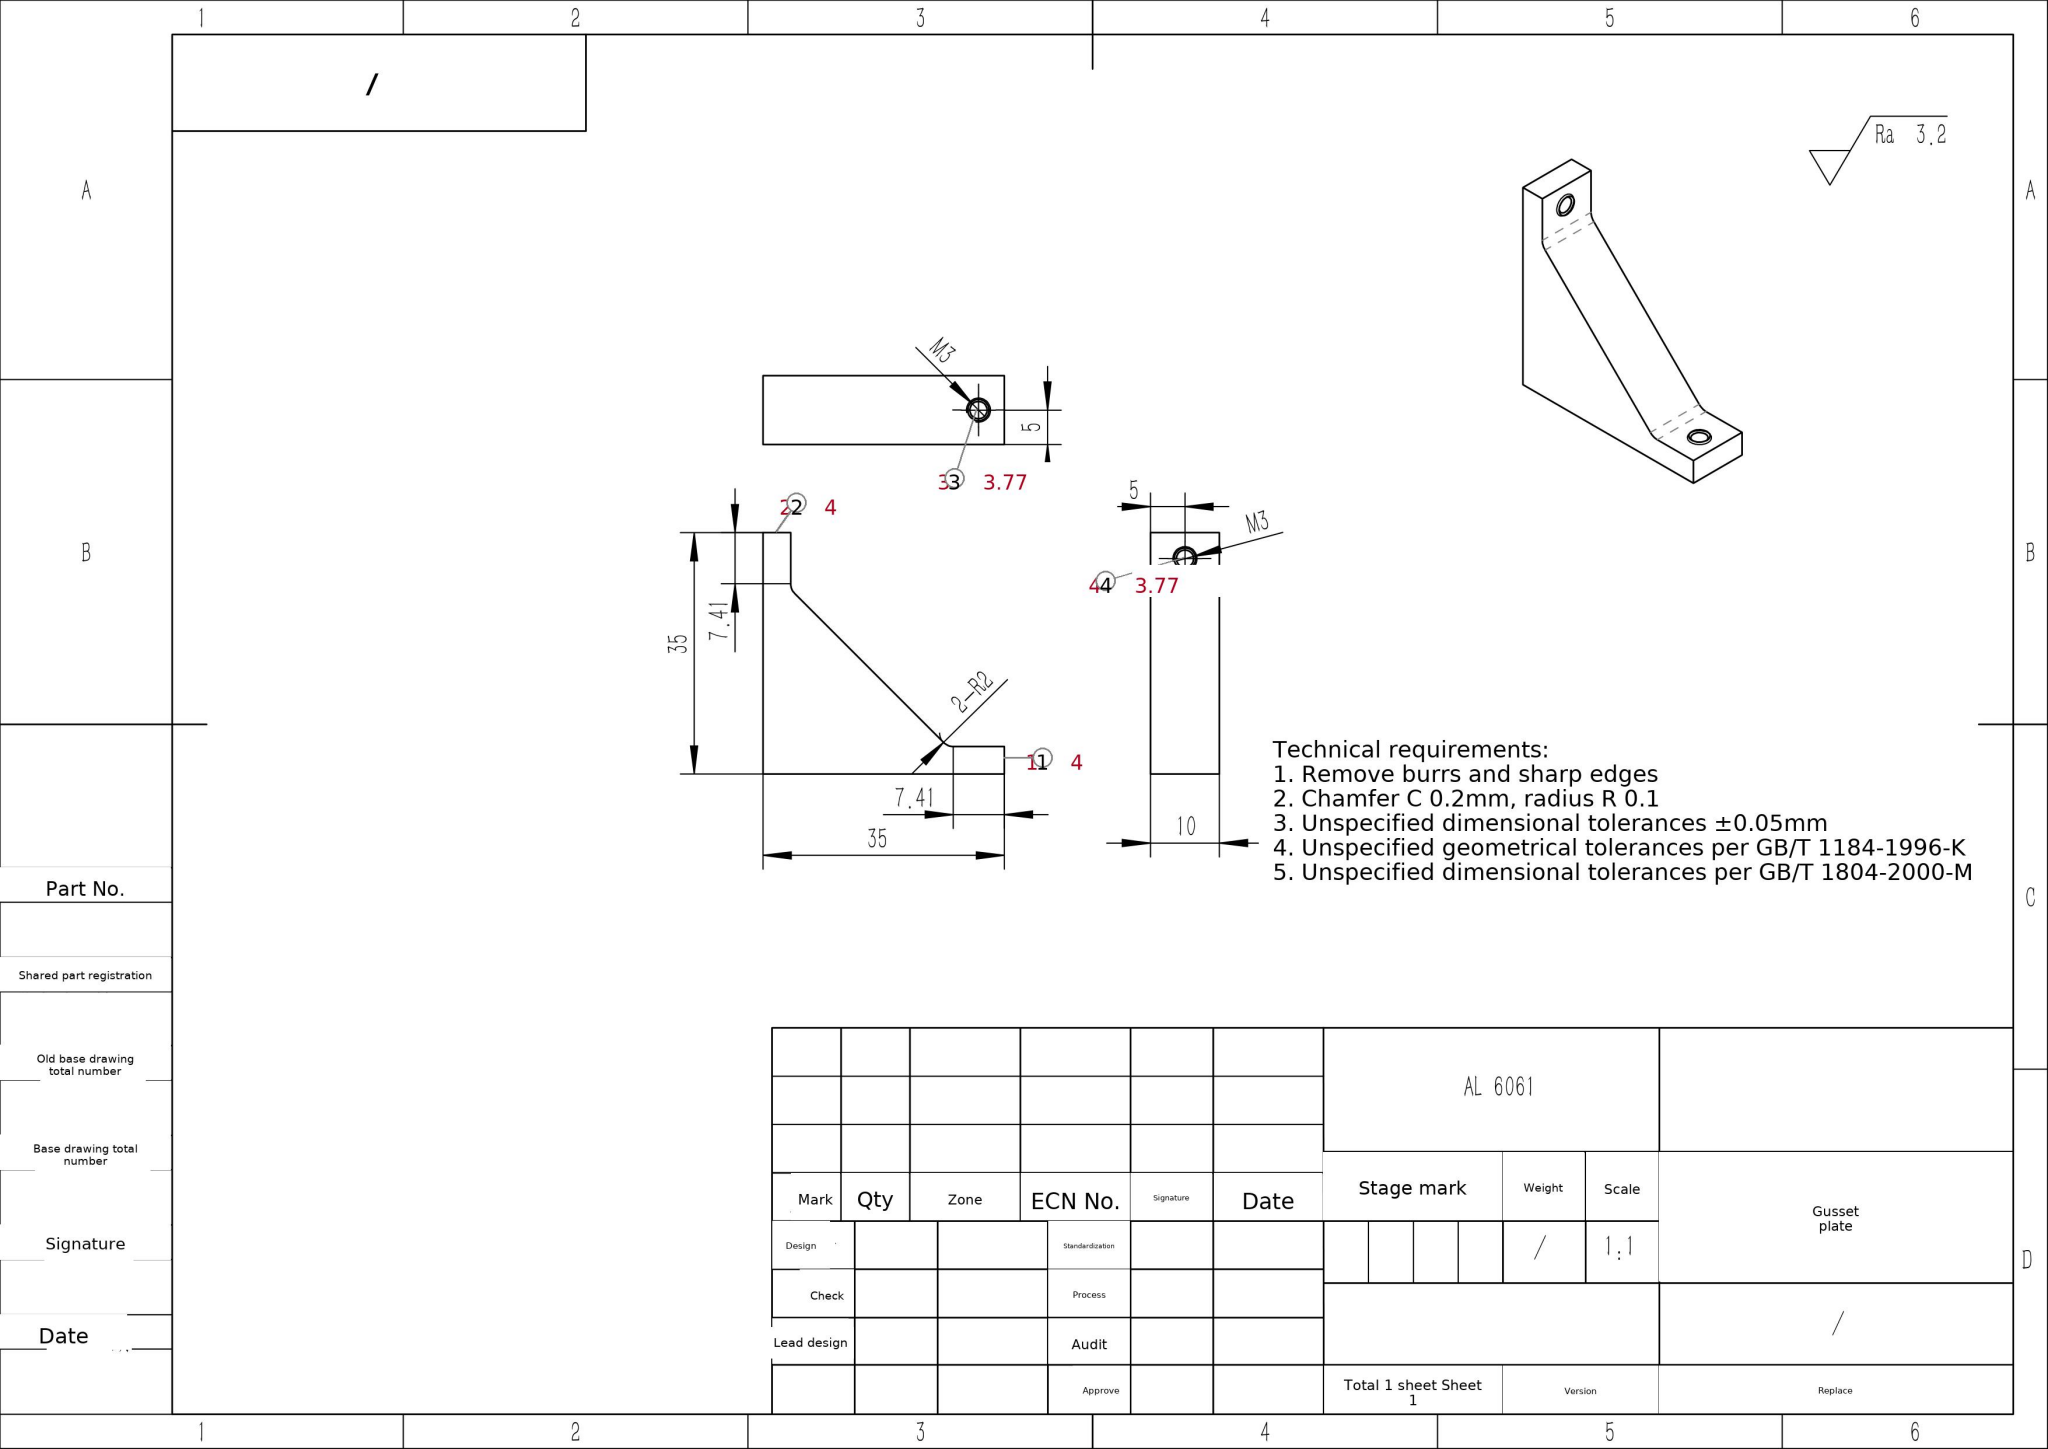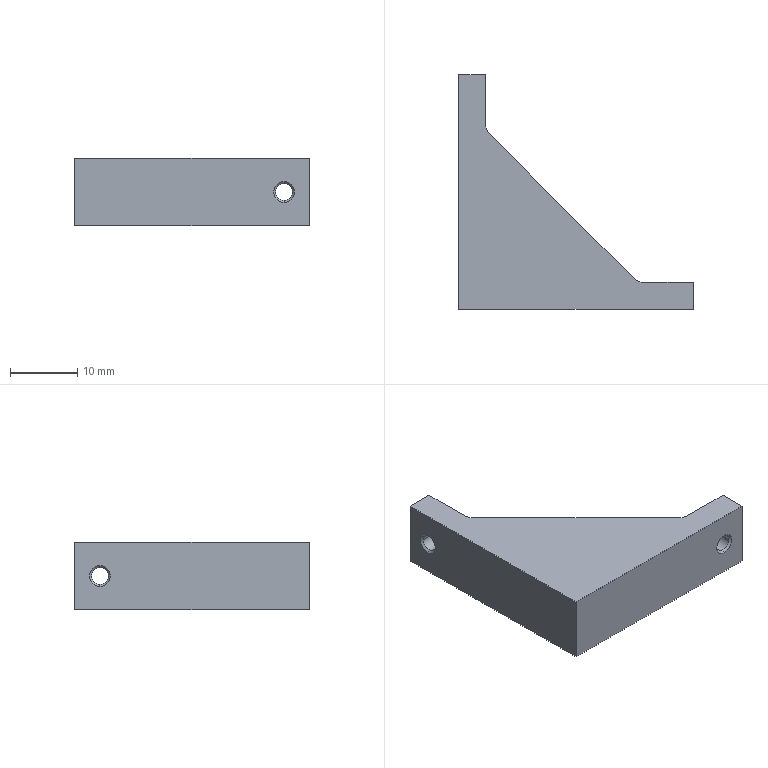Part | SolidWorks | mm | material AL 6061 | 1 solid | 23 faces | box 35 x 35 x 10 mm | volume 5190 mm3 | plane 9 | cone 8 | cylinder 6 | commonest cylinder face diameters 2.5 x4 4 x2
STEP:
#1=CARTESIAN_POINT('',(3.7,31.232,6.25));
#2=VERTEX_POINT('',#1);
#3=CARTESIAN_POINT('',(3.7,29.982,5.));
#4=VERTEX_POINT('',#3);
#5=CARTESIAN_POINT('',(3.7,31.232,5.));
#6=DIRECTION('',(1.,0.,0.));
#7=DIRECTION('',(0.,0.,1.));
#8=AXIS2_PLACEMENT_3D('',#5,#6,#7);
#9=CIRCLE('',#8,1.25);
#10=EDGE_CURVE('',#2,#4,#9,.T.);
#11=ORIENTED_EDGE('',*,*,#10,.F.);
#12=CARTESIAN_POINT('',(4.,31.232,6.55));
#13=VERTEX_POINT('',#12);
#14=CARTESIAN_POINT('',(3.7,31.232,6.25));
#15=DIRECTION('',(0.7071,0.,0.7071));
#16=VECTOR('',#15,1000.);
#17=LINE('',#14,#16);
#18=EDGE_CURVE('',#2,#13,#17,.T.);
#19=ORIENTED_EDGE('',*,*,#18,.T.);
#20=CARTESIAN_POINT('',(4.,31.232,3.45));
#21=VERTEX_POINT('',#20);
#22=CARTESIAN_POINT('',(4.,31.232,5.));
#23=DIRECTION('',(-1.,-0.,0.));
#24=DIRECTION('',(0.,-1.,0.));
#25=AXIS2_PLACEMENT_3D('',#22,#23,#24);
#26=CIRCLE('',#25,1.55);
#27=EDGE_CURVE('',#21,#13,#26,.T.);
#28=ORIENTED_EDGE('',*,*,#27,.F.);
#29=CARTESIAN_POINT('',(3.7,31.232,3.75));
#30=VERTEX_POINT('',#29);
#31=CARTESIAN_POINT('',(3.7,31.232,3.75));
#32=DIRECTION('',(0.7071,0.,-0.7071));
#33=VECTOR('',#32,1000.);
#34=LINE('',#31,#33);
#35=EDGE_CURVE('',#30,#21,#34,.T.);
#36=ORIENTED_EDGE('',*,*,#35,.F.);
#37=CARTESIAN_POINT('',(3.7,31.232,5.));
#38=DIRECTION('',(1.,0.,0.));
#39=DIRECTION('',(0.,0.,1.));
#40=AXIS2_PLACEMENT_3D('',#37,#38,#39);
#41=CIRCLE('',#40,1.25);
#42=EDGE_CURVE('',#4,#30,#41,.T.);
#43=ORIENTED_EDGE('',*,*,#42,.F.);
#44=EDGE_LOOP('',(#11,#19,#28,#36,#43));
#45=FACE_OUTER_BOUND('',#44,.T.);
#46=CARTESIAN_POINT('',(3.7,31.232,5.));
#47=DIRECTION('',(1.,0.,0.));
#48=DIRECTION('',(0.,0.,-1.));
#49=AXIS2_PLACEMENT_3D('',#46,#47,#48);
#50=CONICAL_SURFACE('',#49,1.25,0.7854);
#51=ADVANCED_FACE('',(#45),#50,.F.);
#52=CARTESIAN_POINT('',(0.3,31.232,3.75));
#53=VERTEX_POINT('',#52);
#54=CARTESIAN_POINT('',(0.3,29.982,5.));
#55=VERTEX_POINT('',#54);
#56=CARTESIAN_POINT('',(0.3,31.232,5.));
#57=DIRECTION('',(-1.,0.,0.));
#58=DIRECTION('',(0.,0.,-1.));
#59=AXIS2_PLACEMENT_3D('',#56,#57,#58);
#60=CIRCLE('',#59,1.25);
#61=EDGE_CURVE('',#53,#55,#60,.T.);
#62=ORIENTED_EDGE('',*,*,#61,.F.);
#63=CARTESIAN_POINT('',(0.,31.232,3.45));
#64=VERTEX_POINT('',#63);
#65=CARTESIAN_POINT('',(0.,31.232,3.45));
#66=DIRECTION('',(-0.7071,0.,-0.7071));
#67=VECTOR('',#66,1000.);
#68=LINE('',#65,#67);
#69=EDGE_CURVE('',#53,#64,#68,.T.);
#70=ORIENTED_EDGE('',*,*,#69,.T.);
#71=CARTESIAN_POINT('',(0.,31.232,6.55));
#72=VERTEX_POINT('',#71);
#73=CARTESIAN_POINT('',(0.,31.232,5.));
#74=DIRECTION('',(1.,0.,0.));
#75=DIRECTION('',(0.,0.,-1.));
#76=AXIS2_PLACEMENT_3D('',#73,#74,#75);
#77=CIRCLE('',#76,1.55);
#78=EDGE_CURVE('',#72,#64,#77,.T.);
#79=ORIENTED_EDGE('',*,*,#78,.F.);
#80=CARTESIAN_POINT('',(0.3,31.232,6.25));
#81=VERTEX_POINT('',#80);
#82=CARTESIAN_POINT('',(0.,31.232,6.55));
#83=DIRECTION('',(-0.7071,0.,0.7071));
#84=VECTOR('',#83,1000.);
#85=LINE('',#82,#84);
#86=EDGE_CURVE('',#81,#72,#85,.T.);
#87=ORIENTED_EDGE('',*,*,#86,.F.);
#88=CARTESIAN_POINT('',(0.3,31.232,5.));
#89=DIRECTION('',(-1.,0.,0.));
#90=DIRECTION('',(0.,0.,-1.));
#91=AXIS2_PLACEMENT_3D('',#88,#89,#90);
#92=CIRCLE('',#91,1.25);
#93=EDGE_CURVE('',#55,#81,#92,.T.);
#94=ORIENTED_EDGE('',*,*,#93,.F.);
#95=EDGE_LOOP('',(#62,#70,#79,#87,#94));
#96=FACE_OUTER_BOUND('',#95,.T.);
#97=CARTESIAN_POINT('',(0.,31.232,5.));
#98=DIRECTION('',(-1.,0.,0.));
#99=DIRECTION('',(0.,0.,1.));
#100=AXIS2_PLACEMENT_3D('',#97,#98,#99);
#101=CONICAL_SURFACE('',#100,1.55,0.7854);
#102=ADVANCED_FACE('',(#96),#101,.F.);
#103=CARTESIAN_POINT('',(31.232,3.7,3.75));
#104=VERTEX_POINT('',#103);
#105=CARTESIAN_POINT('',(29.982,3.7,5.));
#106=VERTEX_POINT('',#105);
#107=CARTESIAN_POINT('',(31.232,3.7,5.));
#108=DIRECTION('',(0.,1.,0.));
#109=DIRECTION('',(0.,0.,-1.));
#110=AXIS2_PLACEMENT_3D('',#107,#108,#109);
#111=CIRCLE('',#110,1.25);
#112=EDGE_CURVE('',#104,#106,#111,.T.);
#113=ORIENTED_EDGE('',*,*,#112,.F.);
#114=CARTESIAN_POINT('',(31.232,4.,3.45));
#115=VERTEX_POINT('',#114);
#116=CARTESIAN_POINT('',(31.232,3.7,3.75));
#117=DIRECTION('',(0.,0.7071,-0.7071));
#118=VECTOR('',#117,1000.);
#119=LINE('',#116,#118);
#120=EDGE_CURVE('',#104,#115,#119,.T.);
#121=ORIENTED_EDGE('',*,*,#120,.T.);
#122=CARTESIAN_POINT('',(31.232,4.,6.55));
#123=VERTEX_POINT('',#122);
#124=CARTESIAN_POINT('',(31.232,4.,5.));
#125=DIRECTION('',(0.,-1.,0.));
#126=DIRECTION('',(1.,0.,0.));
#127=AXIS2_PLACEMENT_3D('',#124,#125,#126);
#128=CIRCLE('',#127,1.55);
#129=EDGE_CURVE('',#123,#115,#128,.T.);
#130=ORIENTED_EDGE('',*,*,#129,.F.);
#131=CARTESIAN_POINT('',(31.232,3.7,6.25));
#132=VERTEX_POINT('',#131);
#133=CARTESIAN_POINT('',(31.232,3.7,6.25));
#134=DIRECTION('',(0.,0.7071,0.7071));
#135=VECTOR('',#134,1000.);
#136=LINE('',#133,#135);
#137=EDGE_CURVE('',#132,#123,#136,.T.);
#138=ORIENTED_EDGE('',*,*,#137,.F.);
#139=CARTESIAN_POINT('',(31.232,3.7,5.));
#140=DIRECTION('',(0.,1.,0.));
#141=DIRECTION('',(0.,0.,-1.));
#142=AXIS2_PLACEMENT_3D('',#139,#140,#141);
#143=CIRCLE('',#142,1.25);
#144=EDGE_CURVE('',#106,#132,#143,.T.);
#145=ORIENTED_EDGE('',*,*,#144,.F.);
#146=EDGE_LOOP('',(#113,#121,#130,#138,#145));
#147=FACE_OUTER_BOUND('',#146,.T.);
#148=CARTESIAN_POINT('',(31.232,3.7,5.));
#149=DIRECTION('',(0.,1.,0.));
#150=DIRECTION('',(0.,0.,1.));
#151=AXIS2_PLACEMENT_3D('',#148,#149,#150);
#152=CONICAL_SURFACE('',#151,1.25,0.7854);
#153=ADVANCED_FACE('',(#147),#152,.F.);
#154=CARTESIAN_POINT('',(31.232,0.3,6.25));
#155=VERTEX_POINT('',#154);
#156=CARTESIAN_POINT('',(29.982,0.3,5.));
#157=VERTEX_POINT('',#156);
#158=CARTESIAN_POINT('',(31.232,0.3,5.));
#159=DIRECTION('',(0.,-1.,0.));
#160=DIRECTION('',(0.,0.,1.));
#161=AXIS2_PLACEMENT_3D('',#158,#159,#160);
#162=CIRCLE('',#161,1.25);
#163=EDGE_CURVE('',#155,#157,#162,.T.);
#164=ORIENTED_EDGE('',*,*,#163,.F.);
#165=CARTESIAN_POINT('',(31.232,0.,6.55));
#166=VERTEX_POINT('',#165);
#167=CARTESIAN_POINT('',(31.232,0.,6.55));
#168=DIRECTION('',(0.,-0.7071,0.7071));
#169=VECTOR('',#168,1000.);
#170=LINE('',#167,#169);
#171=EDGE_CURVE('',#155,#166,#170,.T.);
#172=ORIENTED_EDGE('',*,*,#171,.T.);
#173=CARTESIAN_POINT('',(31.232,0.,3.45));
#174=VERTEX_POINT('',#173);
#175=CARTESIAN_POINT('',(31.232,0.,5.));
#176=DIRECTION('',(-0.,1.,0.));
#177=DIRECTION('',(-1.,-0.,0.));
#178=AXIS2_PLACEMENT_3D('',#175,#176,#177);
#179=CIRCLE('',#178,1.55);
#180=EDGE_CURVE('',#174,#166,#179,.T.);
#181=ORIENTED_EDGE('',*,*,#180,.F.);
#182=CARTESIAN_POINT('',(31.232,0.3,3.75));
#183=VERTEX_POINT('',#182);
#184=CARTESIAN_POINT('',(31.232,0.,3.45));
#185=DIRECTION('',(0.,-0.7071,-0.7071));
#186=VECTOR('',#185,1000.);
#187=LINE('',#184,#186);
#188=EDGE_CURVE('',#183,#174,#187,.T.);
#189=ORIENTED_EDGE('',*,*,#188,.F.);
#190=CARTESIAN_POINT('',(31.232,0.3,5.));
#191=DIRECTION('',(0.,-1.,0.));
#192=DIRECTION('',(0.,0.,1.));
#193=AXIS2_PLACEMENT_3D('',#190,#191,#192);
#194=CIRCLE('',#193,1.25);
#195=EDGE_CURVE('',#157,#183,#194,.T.);
#196=ORIENTED_EDGE('',*,*,#195,.F.);
#197=EDGE_LOOP('',(#164,#172,#181,#189,#196));
#198=FACE_OUTER_BOUND('',#197,.T.);
#199=CARTESIAN_POINT('',(31.232,0.,5.));
#200=DIRECTION('',(0.,-1.,0.));
#201=DIRECTION('',(0.,0.,-1.));
#202=AXIS2_PLACEMENT_3D('',#199,#200,#201);
#203=CONICAL_SURFACE('',#202,1.55,0.7854);
#204=ADVANCED_FACE('',(#198),#203,.F.);
#205=CARTESIAN_POINT('',(0.3,32.482,5.));
#206=VERTEX_POINT('',#205);
#207=CARTESIAN_POINT('',(0.3,31.232,5.));
#208=DIRECTION('',(-1.,0.,0.));
#209=DIRECTION('',(0.,0.,-1.));
#210=AXIS2_PLACEMENT_3D('',#207,#208,#209);
#211=CIRCLE('',#210,1.25);
#212=EDGE_CURVE('',#206,#53,#211,.T.);
#213=ORIENTED_EDGE('',*,*,#212,.T.);
#214=ORIENTED_EDGE('',*,*,#61,.T.);
#215=CARTESIAN_POINT('',(-0.,29.982,5.));
#216=DIRECTION('',(1.,0.,0.));
#217=VECTOR('',#216,1000.);
#218=LINE('',#215,#217);
#219=EDGE_CURVE('',#55,#4,#218,.T.);
#220=ORIENTED_EDGE('',*,*,#219,.T.);
#221=ORIENTED_EDGE('',*,*,#42,.T.);
#222=CARTESIAN_POINT('',(3.7,32.482,5.));
#223=VERTEX_POINT('',#222);
#224=CARTESIAN_POINT('',(3.7,31.232,5.));
#225=DIRECTION('',(1.,0.,0.));
#226=DIRECTION('',(0.,0.,1.));
#227=AXIS2_PLACEMENT_3D('',#224,#225,#226);
#228=CIRCLE('',#227,1.25);
#229=EDGE_CURVE('',#30,#223,#228,.T.);
#230=ORIENTED_EDGE('',*,*,#229,.T.);
#231=CARTESIAN_POINT('',(-0.,32.482,5.));
#232=DIRECTION('',(1.,0.,0.));
#233=VECTOR('',#232,1000.);
#234=LINE('',#231,#233);
#235=EDGE_CURVE('',#206,#223,#234,.T.);
#236=ORIENTED_EDGE('',*,*,#235,.F.);
#237=EDGE_LOOP('',(#213,#214,#220,#221,#230,#236));
#238=FACE_OUTER_BOUND('',#237,.T.);
#239=CARTESIAN_POINT('',(-0.,31.232,5.));
#240=DIRECTION('',(1.,0.,0.));
#241=DIRECTION('',(-0.,1.,0.));
#242=AXIS2_PLACEMENT_3D('',#239,#240,#241);
#243=CYLINDRICAL_SURFACE('',#242,1.25);
#244=ADVANCED_FACE('',(#238),#243,.F.);
#245=ORIENTED_EDGE('',*,*,#195,.T.);
#246=CARTESIAN_POINT('',(32.482,0.3,5.));
#247=VERTEX_POINT('',#246);
#248=CARTESIAN_POINT('',(31.232,0.3,5.));
#249=DIRECTION('',(0.,-1.,0.));
#250=DIRECTION('',(0.,0.,1.));
#251=AXIS2_PLACEMENT_3D('',#248,#249,#250);
#252=CIRCLE('',#251,1.25);
#253=EDGE_CURVE('',#183,#247,#252,.T.);
#254=ORIENTED_EDGE('',*,*,#253,.T.);
#255=CARTESIAN_POINT('',(32.482,3.7,5.));
#256=VERTEX_POINT('',#255);
#257=CARTESIAN_POINT('',(32.482,-0.,5.));
#258=DIRECTION('',(-0.,1.,0.));
#259=VECTOR('',#258,1000.);
#260=LINE('',#257,#259);
#261=EDGE_CURVE('',#247,#256,#260,.T.);
#262=ORIENTED_EDGE('',*,*,#261,.T.);
#263=CARTESIAN_POINT('',(31.232,3.7,5.));
#264=DIRECTION('',(0.,1.,0.));
#265=DIRECTION('',(0.,0.,-1.));
#266=AXIS2_PLACEMENT_3D('',#263,#264,#265);
#267=CIRCLE('',#266,1.25);
#268=EDGE_CURVE('',#256,#104,#267,.T.);
#269=ORIENTED_EDGE('',*,*,#268,.T.);
#270=ORIENTED_EDGE('',*,*,#112,.T.);
#271=CARTESIAN_POINT('',(29.982,-0.,5.));
#272=DIRECTION('',(-0.,1.,0.));
#273=VECTOR('',#272,1000.);
#274=LINE('',#271,#273);
#275=EDGE_CURVE('',#157,#106,#274,.T.);
#276=ORIENTED_EDGE('',*,*,#275,.F.);
#277=EDGE_LOOP('',(#245,#254,#262,#269,#270,#276));
#278=FACE_OUTER_BOUND('',#277,.T.);
#279=CARTESIAN_POINT('',(31.232,-0.,5.));
#280=DIRECTION('',(-0.,1.,0.));
#281=DIRECTION('',(-1.,-0.,0.));
#282=AXIS2_PLACEMENT_3D('',#279,#280,#281);
#283=CYLINDRICAL_SURFACE('',#282,1.25);
#284=ADVANCED_FACE('',(#278),#283,.F.);
#285=ORIENTED_EDGE('',*,*,#180,.T.);
#286=CARTESIAN_POINT('',(31.232,0.,5.));
#287=DIRECTION('',(-0.,1.,0.));
#288=DIRECTION('',(-1.,-0.,0.));
#289=AXIS2_PLACEMENT_3D('',#286,#287,#288);
#290=CIRCLE('',#289,1.55);
#291=EDGE_CURVE('',#166,#174,#290,.T.);
#292=ORIENTED_EDGE('',*,*,#291,.T.);
#293=EDGE_LOOP('',(#285,#292));
#294=FACE_BOUND('',#293,.T.);
#295=CARTESIAN_POINT('',(0.,0.,0.));
#296=VERTEX_POINT('',#295);
#297=CARTESIAN_POINT('',(35.,0.,0.));
#298=VERTEX_POINT('',#297);
#299=CARTESIAN_POINT('',(35.,0.,0.));
#300=DIRECTION('',(1.,0.,0.));
#301=VECTOR('',#300,1000.);
#302=LINE('',#299,#301);
#303=EDGE_CURVE('',#296,#298,#302,.T.);
#304=ORIENTED_EDGE('',*,*,#303,.T.);
#305=CARTESIAN_POINT('',(35.,0.,10.));
#306=VERTEX_POINT('',#305);
#307=CARTESIAN_POINT('',(35.,0.,10.));
#308=DIRECTION('',(0.,0.,-1.));
#309=VECTOR('',#308,1000.);
#310=LINE('',#307,#309);
#311=EDGE_CURVE('',#306,#298,#310,.T.);
#312=ORIENTED_EDGE('',*,*,#311,.F.);
#313=CARTESIAN_POINT('',(0.,0.,10.));
#314=VERTEX_POINT('',#313);
#315=CARTESIAN_POINT('',(35.,0.,10.));
#316=DIRECTION('',(1.,0.,0.));
#317=VECTOR('',#316,1000.);
#318=LINE('',#315,#317);
#319=EDGE_CURVE('',#314,#306,#318,.T.);
#320=ORIENTED_EDGE('',*,*,#319,.F.);
#321=CARTESIAN_POINT('',(0.,0.,10.));
#322=DIRECTION('',(0.,0.,-1.));
#323=VECTOR('',#322,1000.);
#324=LINE('',#321,#323);
#325=EDGE_CURVE('',#314,#296,#324,.T.);
#326=ORIENTED_EDGE('',*,*,#325,.T.);
#327=EDGE_LOOP('',(#304,#312,#320,#326));
#328=FACE_OUTER_BOUND('',#327,.T.);
#329=CARTESIAN_POINT('',(35.,0.,10.));
#330=DIRECTION('',(-0.,1.,0.));
#331=DIRECTION('',(-1.,-0.,0.));
#332=AXIS2_PLACEMENT_3D('',#329,#330,#331);
#333=PLANE('',#332);
#334=ADVANCED_FACE('',(#294,#328),#333,.F.);
#335=CARTESIAN_POINT('',(35.,4.,0.));
#336=VERTEX_POINT('',#335);
#337=CARTESIAN_POINT('',(35.,0.,0.));
#338=DIRECTION('',(0.,1.,0.));
#339=VECTOR('',#338,1000.);
#340=LINE('',#337,#339);
#341=EDGE_CURVE('',#298,#336,#340,.T.);
#342=ORIENTED_EDGE('',*,*,#341,.T.);
#343=CARTESIAN_POINT('',(35.,4.,10.));
#344=VERTEX_POINT('',#343);
#345=CARTESIAN_POINT('',(35.,4.,10.));
#346=DIRECTION('',(0.,0.,-1.));
#347=VECTOR('',#346,1000.);
#348=LINE('',#345,#347);
#349=EDGE_CURVE('',#344,#336,#348,.T.);
#350=ORIENTED_EDGE('',*,*,#349,.F.);
#351=CARTESIAN_POINT('',(35.,0.,10.));
#352=DIRECTION('',(0.,1.,0.));
#353=VECTOR('',#352,1000.);
#354=LINE('',#351,#353);
#355=EDGE_CURVE('',#306,#344,#354,.T.);
#356=ORIENTED_EDGE('',*,*,#355,.F.);
#357=ORIENTED_EDGE('',*,*,#311,.T.);
#358=EDGE_LOOP('',(#342,#350,#356,#357));
#359=FACE_OUTER_BOUND('',#358,.T.);
#360=CARTESIAN_POINT('',(35.,0.,10.));
#361=DIRECTION('',(-1.,0.,0.));
#362=DIRECTION('',(0.,0.,1.));
#363=AXIS2_PLACEMENT_3D('',#360,#361,#362);
#364=PLANE('',#363);
#365=ADVANCED_FACE('',(#359),#364,.F.);
#366=ORIENTED_EDGE('',*,*,#129,.T.);
#367=CARTESIAN_POINT('',(31.232,4.,5.));
#368=DIRECTION('',(0.,-1.,0.));
#369=DIRECTION('',(1.,0.,0.));
#370=AXIS2_PLACEMENT_3D('',#367,#368,#369);
#371=CIRCLE('',#370,1.55);
#372=EDGE_CURVE('',#115,#123,#371,.T.);
#373=ORIENTED_EDGE('',*,*,#372,.T.);
#374=EDGE_LOOP('',(#366,#373));
#375=FACE_BOUND('',#374,.T.);
#376=CARTESIAN_POINT('',(27.586,4.,0.));
#377=VERTEX_POINT('',#376);
#378=CARTESIAN_POINT('',(35.,4.,0.));
#379=DIRECTION('',(-1.,-0.,0.));
#380=VECTOR('',#379,1000.);
#381=LINE('',#378,#380);
#382=EDGE_CURVE('',#336,#377,#381,.T.);
#383=ORIENTED_EDGE('',*,*,#382,.T.);
#384=CARTESIAN_POINT('',(27.586,4.,10.));
#385=VERTEX_POINT('',#384);
#386=CARTESIAN_POINT('',(27.586,4.,10.));
#387=DIRECTION('',(0.,0.,1.));
#388=VECTOR('',#387,1000.);
#389=LINE('',#386,#388);
#390=EDGE_CURVE('',#377,#385,#389,.T.);
#391=ORIENTED_EDGE('',*,*,#390,.T.);
#392=CARTESIAN_POINT('',(35.,4.,10.));
#393=DIRECTION('',(-1.,-0.,0.));
#394=VECTOR('',#393,1000.);
#395=LINE('',#392,#394);
#396=EDGE_CURVE('',#344,#385,#395,.T.);
#397=ORIENTED_EDGE('',*,*,#396,.F.);
#398=ORIENTED_EDGE('',*,*,#349,.T.);
#399=EDGE_LOOP('',(#383,#391,#397,#398));
#400=FACE_OUTER_BOUND('',#399,.T.);
#401=CARTESIAN_POINT('',(35.,4.,10.));
#402=DIRECTION('',(0.,-1.,0.));
#403=DIRECTION('',(1.,0.,0.));
#404=AXIS2_PLACEMENT_3D('',#401,#402,#403);
#405=PLANE('',#404);
#406=ADVANCED_FACE('',(#375,#400),#405,.F.);
#407=CARTESIAN_POINT('',(26.172,4.586,0.));
#408=VERTEX_POINT('',#407);
#409=CARTESIAN_POINT('',(4.586,26.172,0.));
#410=VERTEX_POINT('',#409);
#411=CARTESIAN_POINT('',(1.879,28.879,0.));
#412=DIRECTION('',(-0.7071,0.7071,0.));
#413=VECTOR('',#412,1000.);
#414=LINE('',#411,#413);
#415=EDGE_CURVE('',#408,#410,#414,.T.);
#416=ORIENTED_EDGE('',*,*,#415,.T.);
#417=CARTESIAN_POINT('',(4.586,26.172,10.));
#418=VERTEX_POINT('',#417);
#419=CARTESIAN_POINT('',(4.586,26.172,10.));
#420=DIRECTION('',(0.,0.,1.));
#421=VECTOR('',#420,1000.);
#422=LINE('',#419,#421);
#423=EDGE_CURVE('',#410,#418,#422,.T.);
#424=ORIENTED_EDGE('',*,*,#423,.T.);
#425=CARTESIAN_POINT('',(26.172,4.586,10.));
#426=VERTEX_POINT('',#425);
#427=CARTESIAN_POINT('',(1.879,28.879,10.));
#428=DIRECTION('',(-0.7071,0.7071,0.));
#429=VECTOR('',#428,1000.);
#430=LINE('',#427,#429);
#431=EDGE_CURVE('',#426,#418,#430,.T.);
#432=ORIENTED_EDGE('',*,*,#431,.F.);
#433=CARTESIAN_POINT('',(26.172,4.586,0.));
#434=DIRECTION('',(0.,0.,-1.));
#435=VECTOR('',#434,1000.);
#436=LINE('',#433,#435);
#437=EDGE_CURVE('',#426,#408,#436,.T.);
#438=ORIENTED_EDGE('',*,*,#437,.T.);
#439=EDGE_LOOP('',(#416,#424,#432,#438));
#440=FACE_OUTER_BOUND('',#439,.T.);
#441=CARTESIAN_POINT('',(1.879,28.879,10.));
#442=DIRECTION('',(-0.7071,-0.7071,0.));
#443=DIRECTION('',(0.7071,-0.7071,0.));
#444=AXIS2_PLACEMENT_3D('',#441,#442,#443);
#445=PLANE('',#444);
#446=ADVANCED_FACE('',(#440),#445,.F.);
#447=ORIENTED_EDGE('',*,*,#27,.T.);
#448=CARTESIAN_POINT('',(4.,31.232,5.));
#449=DIRECTION('',(-1.,-0.,0.));
#450=DIRECTION('',(0.,-1.,0.));
#451=AXIS2_PLACEMENT_3D('',#448,#449,#450);
#452=CIRCLE('',#451,1.55);
#453=EDGE_CURVE('',#13,#21,#452,.T.);
#454=ORIENTED_EDGE('',*,*,#453,.T.);
#455=EDGE_LOOP('',(#447,#454));
#456=FACE_BOUND('',#455,.T.);
#457=CARTESIAN_POINT('',(4.,27.586,10.));
#458=VERTEX_POINT('',#457);
#459=CARTESIAN_POINT('',(4.,35.,10.));
#460=VERTEX_POINT('',#459);
#461=CARTESIAN_POINT('',(4.,35.,10.));
#462=DIRECTION('',(-0.,1.,0.));
#463=VECTOR('',#462,1000.);
#464=LINE('',#461,#463);
#465=EDGE_CURVE('',#458,#460,#464,.T.);
#466=ORIENTED_EDGE('',*,*,#465,.F.);
#467=CARTESIAN_POINT('',(4.,27.586,0.));
#468=VERTEX_POINT('',#467);
#469=CARTESIAN_POINT('',(4.,27.586,0.));
#470=DIRECTION('',(0.,0.,-1.));
#471=VECTOR('',#470,1000.);
#472=LINE('',#469,#471);
#473=EDGE_CURVE('',#458,#468,#472,.T.);
#474=ORIENTED_EDGE('',*,*,#473,.T.);
#475=CARTESIAN_POINT('',(4.,35.,0.));
#476=VERTEX_POINT('',#475);
#477=CARTESIAN_POINT('',(4.,35.,0.));
#478=DIRECTION('',(-0.,1.,0.));
#479=VECTOR('',#478,1000.);
#480=LINE('',#477,#479);
#481=EDGE_CURVE('',#468,#476,#480,.T.);
#482=ORIENTED_EDGE('',*,*,#481,.T.);
#483=CARTESIAN_POINT('',(4.,35.,10.));
#484=DIRECTION('',(0.,0.,-1.));
#485=VECTOR('',#484,1000.);
#486=LINE('',#483,#485);
#487=EDGE_CURVE('',#460,#476,#486,.T.);
#488=ORIENTED_EDGE('',*,*,#487,.F.);
#489=EDGE_LOOP('',(#466,#474,#482,#488));
#490=FACE_OUTER_BOUND('',#489,.T.);
#491=CARTESIAN_POINT('',(4.,35.,10.));
#492=DIRECTION('',(-1.,-0.,0.));
#493=DIRECTION('',(0.,-1.,0.));
#494=AXIS2_PLACEMENT_3D('',#491,#492,#493);
#495=PLANE('',#494);
#496=ADVANCED_FACE('',(#456,#490),#495,.F.);
#497=CARTESIAN_POINT('',(0.,35.,0.));
#498=VERTEX_POINT('',#497);
#499=CARTESIAN_POINT('',(0.,35.,0.));
#500=DIRECTION('',(-1.,0.,0.));
#501=VECTOR('',#500,1000.);
#502=LINE('',#499,#501);
#503=EDGE_CURVE('',#476,#498,#502,.T.);
#504=ORIENTED_EDGE('',*,*,#503,.T.);
#505=CARTESIAN_POINT('',(0.,35.,10.));
#506=VERTEX_POINT('',#505);
#507=CARTESIAN_POINT('',(0.,35.,10.));
#508=DIRECTION('',(0.,0.,-1.));
#509=VECTOR('',#508,1000.);
#510=LINE('',#507,#509);
#511=EDGE_CURVE('',#506,#498,#510,.T.);
#512=ORIENTED_EDGE('',*,*,#511,.F.);
#513=CARTESIAN_POINT('',(0.,35.,10.));
#514=DIRECTION('',(-1.,0.,0.));
#515=VECTOR('',#514,1000.);
#516=LINE('',#513,#515);
#517=EDGE_CURVE('',#460,#506,#516,.T.);
#518=ORIENTED_EDGE('',*,*,#517,.F.);
#519=ORIENTED_EDGE('',*,*,#487,.T.);
#520=EDGE_LOOP('',(#504,#512,#518,#519));
#521=FACE_OUTER_BOUND('',#520,.T.);
#522=CARTESIAN_POINT('',(0.,35.,10.));
#523=DIRECTION('',(0.,-1.,0.));
#524=DIRECTION('',(0.,0.,-1.));
#525=AXIS2_PLACEMENT_3D('',#522,#523,#524);
#526=PLANE('',#525);
#527=ADVANCED_FACE('',(#521),#526,.F.);
#528=ORIENTED_EDGE('',*,*,#78,.T.);
#529=CARTESIAN_POINT('',(0.,31.232,5.));
#530=DIRECTION('',(1.,0.,0.));
#531=DIRECTION('',(0.,0.,-1.));
#532=AXIS2_PLACEMENT_3D('',#529,#530,#531);
#533=CIRCLE('',#532,1.55);
#534=EDGE_CURVE('',#64,#72,#533,.T.);
#535=ORIENTED_EDGE('',*,*,#534,.T.);
#536=EDGE_LOOP('',(#528,#535));
#537=FACE_BOUND('',#536,.T.);
#538=CARTESIAN_POINT('',(0.,0.,0.));
#539=DIRECTION('',(0.,-1.,0.));
#540=VECTOR('',#539,1000.);
#541=LINE('',#538,#540);
#542=EDGE_CURVE('',#498,#296,#541,.T.);
#543=ORIENTED_EDGE('',*,*,#542,.T.);
#544=ORIENTED_EDGE('',*,*,#325,.F.);
#545=CARTESIAN_POINT('',(0.,0.,10.));
#546=DIRECTION('',(0.,-1.,0.));
#547=VECTOR('',#546,1000.);
#548=LINE('',#545,#547);
#549=EDGE_CURVE('',#506,#314,#548,.T.);
#550=ORIENTED_EDGE('',*,*,#549,.F.);
#551=ORIENTED_EDGE('',*,*,#511,.T.);
#552=EDGE_LOOP('',(#543,#544,#550,#551));
#553=FACE_OUTER_BOUND('',#552,.T.);
#554=CARTESIAN_POINT('',(0.,0.,10.));
#555=DIRECTION('',(1.,0.,0.));
#556=DIRECTION('',(0.,0.,-1.));
#557=AXIS2_PLACEMENT_3D('',#554,#555,#556);
#558=PLANE('',#557);
#559=ADVANCED_FACE('',(#537,#553),#558,.F.);
#560=ORIENTED_EDGE('',*,*,#319,.T.);
#561=ORIENTED_EDGE('',*,*,#355,.T.);
#562=ORIENTED_EDGE('',*,*,#396,.T.);
#563=CARTESIAN_POINT('',(27.586,6.,10.));
#564=DIRECTION('',(0.,0.,-1.));
#565=DIRECTION('',(-1.,0.,0.));
#566=AXIS2_PLACEMENT_3D('',#563,#564,#565);
#567=CIRCLE('',#566,2.);
#568=EDGE_CURVE('',#385,#426,#567,.T.);
#569=ORIENTED_EDGE('',*,*,#568,.T.);
#570=ORIENTED_EDGE('',*,*,#431,.T.);
#571=CARTESIAN_POINT('',(6.,27.586,10.));
#572=DIRECTION('',(0.,0.,-1.));
#573=DIRECTION('',(-1.,0.,0.));
#574=AXIS2_PLACEMENT_3D('',#571,#572,#573);
#575=CIRCLE('',#574,2.);
#576=EDGE_CURVE('',#418,#458,#575,.T.);
#577=ORIENTED_EDGE('',*,*,#576,.T.);
#578=ORIENTED_EDGE('',*,*,#465,.T.);
#579=ORIENTED_EDGE('',*,*,#517,.T.);
#580=ORIENTED_EDGE('',*,*,#549,.T.);
#581=EDGE_LOOP('',(#560,#561,#562,#569,#570,#577,#578,#579,#580));
#582=FACE_OUTER_BOUND('',#581,.T.);
#583=CARTESIAN_POINT('',(0.,0.,10.));
#584=DIRECTION('',(0.,0.,-1.));
#585=DIRECTION('',(-1.,0.,0.));
#586=AXIS2_PLACEMENT_3D('',#583,#584,#585);
#587=PLANE('',#586);
#588=ADVANCED_FACE('',(#582),#587,.F.);
#589=ORIENTED_EDGE('',*,*,#303,.F.);
#590=ORIENTED_EDGE('',*,*,#542,.F.);
#591=ORIENTED_EDGE('',*,*,#503,.F.);
#592=ORIENTED_EDGE('',*,*,#481,.F.);
#593=CARTESIAN_POINT('',(6.,27.586,0.));
#594=DIRECTION('',(0.,0.,1.));
#595=DIRECTION('',(-1.,0.,0.));
#596=AXIS2_PLACEMENT_3D('',#593,#594,#595);
#597=CIRCLE('',#596,2.);
#598=EDGE_CURVE('',#468,#410,#597,.T.);
#599=ORIENTED_EDGE('',*,*,#598,.T.);
#600=ORIENTED_EDGE('',*,*,#415,.F.);
#601=CARTESIAN_POINT('',(27.586,6.,0.));
#602=DIRECTION('',(0.,0.,1.));
#603=DIRECTION('',(-1.,0.,0.));
#604=AXIS2_PLACEMENT_3D('',#601,#602,#603);
#605=CIRCLE('',#604,2.);
#606=EDGE_CURVE('',#408,#377,#605,.T.);
#607=ORIENTED_EDGE('',*,*,#606,.T.);
#608=ORIENTED_EDGE('',*,*,#382,.F.);
#609=ORIENTED_EDGE('',*,*,#341,.F.);
#610=EDGE_LOOP('',(#589,#590,#591,#592,#599,#600,#607,#608,#609));
#611=FACE_OUTER_BOUND('',#610,.T.);
#612=CARTESIAN_POINT('',(0.,0.,0.));
#613=DIRECTION('',(0.,0.,-1.));
#614=DIRECTION('',(-1.,0.,0.));
#615=AXIS2_PLACEMENT_3D('',#612,#613,#614);
#616=PLANE('',#615);
#617=ADVANCED_FACE('',(#611),#616,.T.);
#618=ORIENTED_EDGE('',*,*,#261,.F.);
#619=CARTESIAN_POINT('',(31.232,0.3,5.));
#620=DIRECTION('',(0.,-1.,0.));
#621=DIRECTION('',(0.,0.,1.));
#622=AXIS2_PLACEMENT_3D('',#619,#620,#621);
#623=CIRCLE('',#622,1.25);
#624=EDGE_CURVE('',#247,#155,#623,.T.);
#625=ORIENTED_EDGE('',*,*,#624,.T.);
#626=ORIENTED_EDGE('',*,*,#163,.T.);
#627=ORIENTED_EDGE('',*,*,#275,.T.);
#628=ORIENTED_EDGE('',*,*,#144,.T.);
#629=CARTESIAN_POINT('',(31.232,3.7,5.));
#630=DIRECTION('',(0.,1.,0.));
#631=DIRECTION('',(0.,0.,-1.));
#632=AXIS2_PLACEMENT_3D('',#629,#630,#631);
#633=CIRCLE('',#632,1.25);
#634=EDGE_CURVE('',#132,#256,#633,.T.);
#635=ORIENTED_EDGE('',*,*,#634,.T.);
#636=EDGE_LOOP('',(#618,#625,#626,#627,#628,#635));
#637=FACE_OUTER_BOUND('',#636,.T.);
#638=CARTESIAN_POINT('',(31.232,-0.,5.));
#639=DIRECTION('',(-0.,1.,0.));
#640=DIRECTION('',(-1.,-0.,0.));
#641=AXIS2_PLACEMENT_3D('',#638,#639,#640);
#642=CYLINDRICAL_SURFACE('',#641,1.25);
#643=ADVANCED_FACE('',(#637),#642,.F.);
#644=ORIENTED_EDGE('',*,*,#219,.F.);
#645=ORIENTED_EDGE('',*,*,#93,.T.);
#646=CARTESIAN_POINT('',(0.3,31.232,5.));
#647=DIRECTION('',(-1.,0.,0.));
#648=DIRECTION('',(0.,0.,-1.));
#649=AXIS2_PLACEMENT_3D('',#646,#647,#648);
#650=CIRCLE('',#649,1.25);
#651=EDGE_CURVE('',#81,#206,#650,.T.);
#652=ORIENTED_EDGE('',*,*,#651,.T.);
#653=ORIENTED_EDGE('',*,*,#235,.T.);
#654=CARTESIAN_POINT('',(3.7,31.232,5.));
#655=DIRECTION('',(1.,0.,0.));
#656=DIRECTION('',(0.,0.,1.));
#657=AXIS2_PLACEMENT_3D('',#654,#655,#656);
#658=CIRCLE('',#657,1.25);
#659=EDGE_CURVE('',#223,#2,#658,.T.);
#660=ORIENTED_EDGE('',*,*,#659,.T.);
#661=ORIENTED_EDGE('',*,*,#10,.T.);
#662=EDGE_LOOP('',(#644,#645,#652,#653,#660,#661));
#663=FACE_OUTER_BOUND('',#662,.T.);
#664=CARTESIAN_POINT('',(-0.,31.232,5.));
#665=DIRECTION('',(1.,0.,0.));
#666=DIRECTION('',(-0.,1.,0.));
#667=AXIS2_PLACEMENT_3D('',#664,#665,#666);
#668=CYLINDRICAL_SURFACE('',#667,1.25);
#669=ADVANCED_FACE('',(#663),#668,.F.);
#670=ORIENTED_EDGE('',*,*,#171,.F.);
#671=ORIENTED_EDGE('',*,*,#624,.F.);
#672=ORIENTED_EDGE('',*,*,#253,.F.);
#673=ORIENTED_EDGE('',*,*,#188,.T.);
#674=ORIENTED_EDGE('',*,*,#291,.F.);
#675=EDGE_LOOP('',(#670,#671,#672,#673,#674));
#676=FACE_OUTER_BOUND('',#675,.T.);
#677=CARTESIAN_POINT('',(31.232,0.,5.));
#678=DIRECTION('',(0.,-1.,0.));
#679=DIRECTION('',(0.,0.,-1.));
#680=AXIS2_PLACEMENT_3D('',#677,#678,#679);
#681=CONICAL_SURFACE('',#680,1.55,0.7854);
#682=ADVANCED_FACE('',(#676),#681,.F.);
#683=ORIENTED_EDGE('',*,*,#120,.F.);
#684=ORIENTED_EDGE('',*,*,#268,.F.);
#685=ORIENTED_EDGE('',*,*,#634,.F.);
#686=ORIENTED_EDGE('',*,*,#137,.T.);
#687=ORIENTED_EDGE('',*,*,#372,.F.);
#688=EDGE_LOOP('',(#683,#684,#685,#686,#687));
#689=FACE_OUTER_BOUND('',#688,.T.);
#690=CARTESIAN_POINT('',(31.232,3.7,5.));
#691=DIRECTION('',(0.,1.,0.));
#692=DIRECTION('',(0.,0.,1.));
#693=AXIS2_PLACEMENT_3D('',#690,#691,#692);
#694=CONICAL_SURFACE('',#693,1.25,0.7854);
#695=ADVANCED_FACE('',(#689),#694,.F.);
#696=ORIENTED_EDGE('',*,*,#69,.F.);
#697=ORIENTED_EDGE('',*,*,#212,.F.);
#698=ORIENTED_EDGE('',*,*,#651,.F.);
#699=ORIENTED_EDGE('',*,*,#86,.T.);
#700=ORIENTED_EDGE('',*,*,#534,.F.);
#701=EDGE_LOOP('',(#696,#697,#698,#699,#700));
#702=FACE_OUTER_BOUND('',#701,.T.);
#703=CARTESIAN_POINT('',(0.,31.232,5.));
#704=DIRECTION('',(-1.,0.,0.));
#705=DIRECTION('',(0.,0.,1.));
#706=AXIS2_PLACEMENT_3D('',#703,#704,#705);
#707=CONICAL_SURFACE('',#706,1.55,0.7854);
#708=ADVANCED_FACE('',(#702),#707,.F.);
#709=ORIENTED_EDGE('',*,*,#18,.F.);
#710=ORIENTED_EDGE('',*,*,#659,.F.);
#711=ORIENTED_EDGE('',*,*,#229,.F.);
#712=ORIENTED_EDGE('',*,*,#35,.T.);
#713=ORIENTED_EDGE('',*,*,#453,.F.);
#714=EDGE_LOOP('',(#709,#710,#711,#712,#713));
#715=FACE_OUTER_BOUND('',#714,.T.);
#716=CARTESIAN_POINT('',(3.7,31.232,5.));
#717=DIRECTION('',(1.,0.,0.));
#718=DIRECTION('',(0.,0.,-1.));
#719=AXIS2_PLACEMENT_3D('',#716,#717,#718);
#720=CONICAL_SURFACE('',#719,1.25,0.7854);
#721=ADVANCED_FACE('',(#715),#720,.F.);
#722=ORIENTED_EDGE('',*,*,#576,.F.);
#723=ORIENTED_EDGE('',*,*,#423,.F.);
#724=ORIENTED_EDGE('',*,*,#598,.F.);
#725=ORIENTED_EDGE('',*,*,#473,.F.);
#726=EDGE_LOOP('',(#722,#723,#724,#725));
#727=FACE_OUTER_BOUND('',#726,.T.);
#728=CARTESIAN_POINT('',(6.,27.586,10.));
#729=DIRECTION('',(0.,0.,1.));
#730=DIRECTION('',(1.,0.,0.));
#731=AXIS2_PLACEMENT_3D('',#728,#729,#730);
#732=CYLINDRICAL_SURFACE('',#731,2.);
#733=ADVANCED_FACE('',(#727),#732,.F.);
#734=ORIENTED_EDGE('',*,*,#568,.F.);
#735=ORIENTED_EDGE('',*,*,#390,.F.);
#736=ORIENTED_EDGE('',*,*,#606,.F.);
#737=ORIENTED_EDGE('',*,*,#437,.F.);
#738=EDGE_LOOP('',(#734,#735,#736,#737));
#739=FACE_OUTER_BOUND('',#738,.T.);
#740=CARTESIAN_POINT('',(27.586,6.,10.));
#741=DIRECTION('',(0.,0.,1.));
#742=DIRECTION('',(1.,0.,0.));
#743=AXIS2_PLACEMENT_3D('',#740,#741,#742);
#744=CYLINDRICAL_SURFACE('',#743,2.);
#745=ADVANCED_FACE('',(#739),#744,.F.);
#746=CLOSED_SHELL('',(#51,#102,#153,#204,#244,#284,#334,#365,#406,#446,#496,#527,#559,#588,#617,#643,#669,#682,#695,#708,#721,#733,#745));
#747=MANIFOLD_SOLID_BREP('',#746);
#748=CARTESIAN_POINT('',(0.,0.,0.));
#749=DIRECTION('',(0.,0.,1.));
#750=DIRECTION('',(1.,0.,0.));
#751=AXIS2_PLACEMENT_3D('',#748,#749,#750);
#752=(LENGTH_UNIT()NAMED_UNIT(*)SI_UNIT(.MILLI.,.METRE.));
#753=UNCERTAINTY_MEASURE_WITH_UNIT(LENGTH_MEASURE(0.00001),#752,'','');
#754=(NAMED_UNIT(*)PLANE_ANGLE_UNIT()SI_UNIT($,.RADIAN.));
#755=(NAMED_UNIT(*)SI_UNIT($,.STERADIAN.)SOLID_ANGLE_UNIT());
#756=(GEOMETRIC_REPRESENTATION_CONTEXT(3)GLOBAL_UNCERTAINTY_ASSIGNED_CONTEXT((#753))GLOBAL_UNIT_ASSIGNED_CONTEXT((#752,#754,#755))REPRESENTATION_CONTEXT('',''));
#757=ADVANCED_BREP_SHAPE_REPRESENTATION('',(#747,#751),#756);